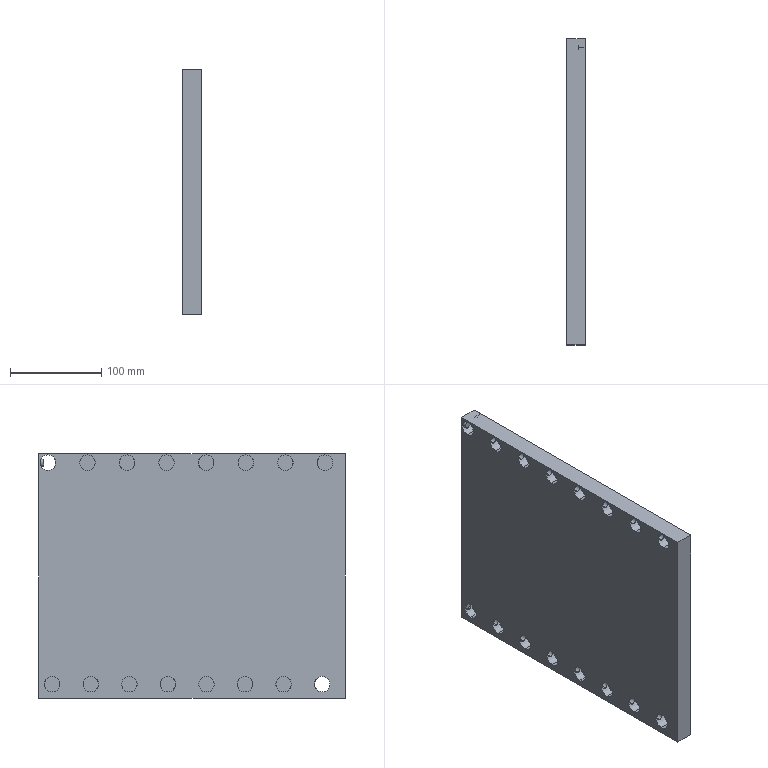Component | SolidWorks | HeatExchangePlate-1_PlateOne-1 | 1 solid | 92 faces | box 20 x 334.74 x 267.35 mm | volume 1729859 mm3 | cylinder 68 | plane 24 | commonest cylinder face diameters 17 x32 8 x16 8.001 x16 18.9 x4
build123d program:
from build123d import *

# Parameters (mm, degrees)
SKETCH1_2_R         = 8.5
BOSS_EXTRUDE1_DEPTH = 20
SKETCH2_R           = 8.892
SKETCH2_R_2         = 8.5
BOSS_EXTRUDE2_DEPTH = 10
SKETCH5_R           = 4.001
SKETCH5_R_2         = 4
CUT_EXTRUDE2_DEPTH  = 314
SKETCH6_R           = 4.001
SKETCH6_R_2         = 4
BOSS_EXTRUDE3_DEPTH = 5
SKETCH1_R           = 9.45
CUT_EXTRUDE1_DEPTH  = 7.6


with BuildPart() as part:
    # Sketch1_2 → Boss-Extrude1 (new body)
    with BuildSketch(Plane.XY):
        Polygon((-51.011, -555.291), (-51.011, -560.907), (-318.362, -560.907), (-318.362, -226.167), (-312.688, -226.167), (-51.011, -226.167), align=None)
        with Locations(Location((-60.761, -235.917, 0), (0, 0, 180))):
            Circle(SKETCH1_2_R, mode=Mode.SUBTRACT)
        with Locations((-303.011, -535.907)):
            Circle(SKETCH1_2_R, mode=Mode.SUBTRACT)
        with Locations(Location((-60.761, -279.197, 0), (0, 0, 180))):
            Circle(SKETCH1_2_R, mode=Mode.SUBTRACT)
        with Locations(Location((-60.761, -322.477, 0), (0, 0, 180))):
            Circle(SKETCH1_2_R, mode=Mode.SUBTRACT)
        with Locations(Location((-60.761, -365.757, 0), (0, 0, 180))):
            Circle(SKETCH1_2_R, mode=Mode.SUBTRACT)
        with Locations(Location((-60.761, -409.037, 0), (0, 0, 180))):
            Circle(SKETCH1_2_R, mode=Mode.SUBTRACT)
        with Locations(Location((-60.761, -452.317, 0), (0, 0, 180))):
            Circle(SKETCH1_2_R, mode=Mode.SUBTRACT)
        with Locations(Location((-60.761, -495.597, 0), (0, 0, 180))):
            Circle(SKETCH1_2_R, mode=Mode.SUBTRACT)
        with Locations(Location((-60.761, -538.877, 0), (0, 0, 180))):
            Circle(SKETCH1_2_R, mode=Mode.SUBTRACT)
        with Locations((-303.011, -493.727)):
            Circle(SKETCH1_2_R, mode=Mode.SUBTRACT)
        with Locations((-303.011, -451.547)):
            Circle(SKETCH1_2_R, mode=Mode.SUBTRACT)
        with Locations((-303.011, -409.367)):
            Circle(SKETCH1_2_R, mode=Mode.SUBTRACT)
        with Locations((-303.011, -367.187)):
            Circle(SKETCH1_2_R, mode=Mode.SUBTRACT)
        with Locations((-303.011, -325.007)):
            Circle(SKETCH1_2_R, mode=Mode.SUBTRACT)
        with Locations((-303.011, -282.827)):
            Circle(SKETCH1_2_R, mode=Mode.SUBTRACT)
        with Locations((-303.011, -240.647)):
            Circle(SKETCH1_2_R, mode=Mode.SUBTRACT)
    extrude(amount=BOSS_EXTRUDE1_DEPTH)

    # Sketch2 → Boss-Extrude2 (add)
    with BuildSketch(Plane(origin=(0, 0, 0), x_dir=(-1, 0, 0), z_dir=(0, 0, -1))):
        with Locations((60.761, -538.877)):
            Circle(SKETCH2_R)
        with Locations((303.011, -493.727)):
            Circle(SKETCH2_R_2)
        with Locations((60.761, -495.597)):
            Circle(SKETCH2_R_2)
        with Locations((303.011, -451.547)):
            Circle(SKETCH2_R_2)
        with Locations((303.011, -409.367)):
            Circle(SKETCH2_R_2)
        with Locations((303.011, -367.187)):
            Circle(SKETCH2_R_2)
        with Locations((303.011, -325.007)):
            Circle(SKETCH2_R_2)
        with Locations((303.011, -282.827)):
            Circle(SKETCH2_R_2)
        with Locations((303.011, -240.647)):
            Circle(SKETCH2_R_2)
        with Locations((60.761, -452.317)):
            Circle(SKETCH2_R_2)
        with Locations((60.761, -409.037)):
            Circle(SKETCH2_R_2)
        with Locations((60.761, -365.757)):
            Circle(SKETCH2_R_2)
        with Locations((60.761, -322.477)):
            Circle(SKETCH2_R_2)
        with Locations((60.761, -279.197)):
            Circle(SKETCH2_R_2)
    extrude(amount=-BOSS_EXTRUDE2_DEPTH)

    # Sketch5 → Cut-Extrude2 (cut)
    with BuildSketch(Plane(origin=(0, -226.167, 0), x_dir=(1, 0, 0), z_dir=(0, 1, 0))):
        with Locations(Location((-303.012, -15, 0), (0, 0, 180))):
            Circle(SKETCH5_R)
        with Locations(Location((-60.761, -15, 0), (0, 0, 180))):
            Circle(SKETCH5_R_2)
    extrude(amount=-CUT_EXTRUDE2_DEPTH, mode=Mode.SUBTRACT)

    # Sketch6 → Boss-Extrude3 (add)
    with BuildSketch(Plane(origin=(0, -226.167, 0), x_dir=(1, 0, 0), z_dir=(0, 1, 0))):
        with Locations(Location((-303.012, -15, 0), (0, 0, 180))):
            Circle(SKETCH6_R)
        with Locations(Location((-60.761, -15, 0), (0, 0, 180))):
            Circle(SKETCH6_R_2)
    extrude(amount=-BOSS_EXTRUDE3_DEPTH)

    # Sketch1 → Cut-Extrude1 (cut)
    with BuildSketch(Plane(origin=(0, 0, 0), x_dir=(-1, 0, 0), z_dir=(0, 0, -1))):
        with Locations((303.011, -535.907)):
            Circle(SKETCH1_R)
        with Locations((60.761, -235.917)):
            Circle(SKETCH1_R)
    extrude(amount=-CUT_EXTRUDE1_DEPTH, mode=Mode.SUBTRACT)


solid = part.part

# Placed as in the assembly
solid = solid.moved(Location((606.39, 1046.117, 185.762), (0, -90, 0)))